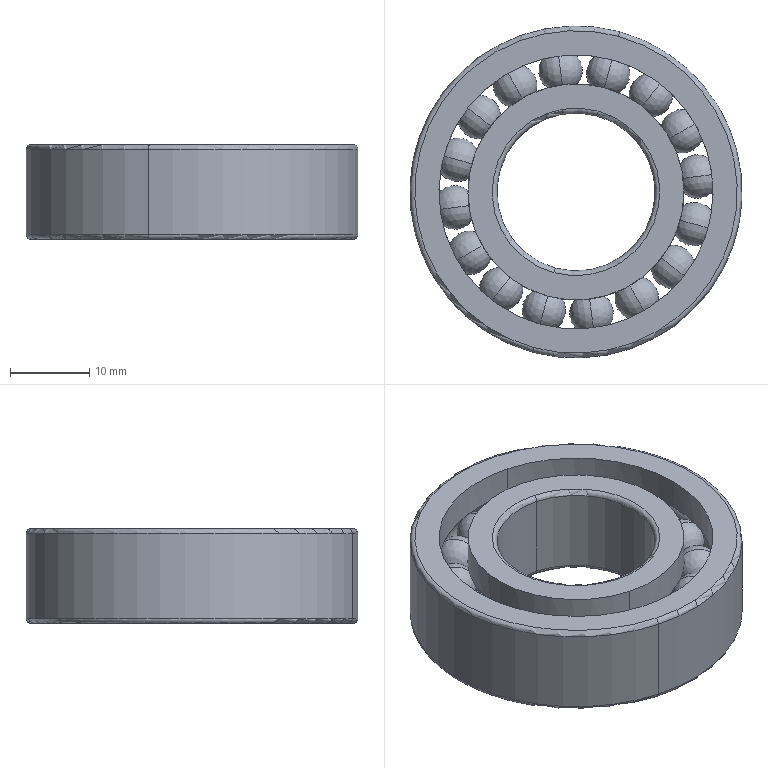Component | SolidWorks | 6004DeepGrooveBallBearing(BG276-94)0-2 | 1 solid | 104 faces | volume 9425 mm3 | torus 56 | sphere 32 | cylinder 12 | plane 4 | commonest cylinder face diameters 27.33 x4 34.67 x4 20 x2 42 x2